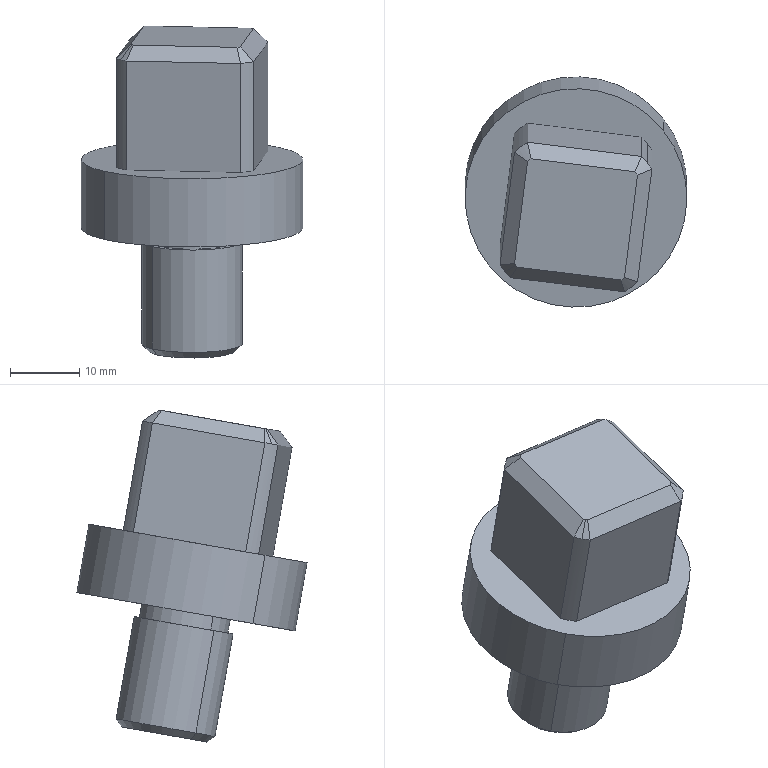Component | SolidWorks | 27PlugScrew-1 | 1 solid | 31 faces | box 32 x 33.25 x 47.93 mm | volume 17888 mm3 | plane 13 | cylinder 11 | cone 7 | commonest cylinder face diameters 26 x5 14.5 x2 13 x2 32 x2
STEP:
#1=COLOUR_RGB('',0.7922,0.8196,0.9333);
#2=FILL_AREA_STYLE_COLOUR('',#1);
#3=FILL_AREA_STYLE('',(#2));
#4=SURFACE_STYLE_FILL_AREA(#3);
#5=SURFACE_SIDE_STYLE('',(#4));
#6=SURFACE_STYLE_USAGE(.BOTH.,#5);
#7=PRESENTATION_STYLE_ASSIGNMENT((#6));
#8=CARTESIAN_POINT('',(2.951,-7.079,23.));
#9=VERTEX_POINT('',#8);
#10=CARTESIAN_POINT('',(3.339,-6.782,23.053));
#11=VERTEX_POINT('',#10);
#12=CARTESIAN_POINT('',(3.145,-6.931,23.027));
#13=DIRECTION('',(-0.,0.1736,-0.9848));
#14=DIRECTION('',(-0.7898,-0.6041,-0.1065));
#15=AXIS2_PLACEMENT_3D('',#12,#13,#14);
#16=CIRCLE('',#15,0.2461);
#17=EDGE_CURVE('',#9,#11,#16,.T.);
#18=ORIENTED_EDGE('',*,*,#17,.F.);
#19=CARTESIAN_POINT('',(2.92,-7.11,23.035));
#20=VERTEX_POINT('',#19);
#21=CARTESIAN_POINT('',(2.951,-7.079,23.));
#22=DIRECTION('',(-0.5585,-0.5499,0.621));
#23=VECTOR('',#22,39.37);
#24=LINE('',#21,#23);
#25=EDGE_CURVE('',#9,#20,#24,.T.);
#26=ORIENTED_EDGE('',*,*,#25,.T.);
#27=CARTESIAN_POINT('',(3.37,-6.765,23.096));
#28=VERTEX_POINT('',#27);
#29=CARTESIAN_POINT('',(3.145,-6.938,23.065));
#30=DIRECTION('',(0.,-0.1736,0.9848));
#31=DIRECTION('',(-0.7898,-0.6041,-0.1065));
#32=AXIS2_PLACEMENT_3D('',#29,#30,#31);
#33=CIRCLE('',#32,0.2854);
#34=EDGE_CURVE('',#28,#20,#33,.T.);
#35=ORIENTED_EDGE('',*,*,#34,.F.);
#36=CARTESIAN_POINT('',(3.339,-6.782,23.053));
#37=DIRECTION('',(0.5585,0.3043,0.7717));
#38=VECTOR('',#37,39.37);
#39=LINE('',#36,#38);
#40=EDGE_CURVE('',#11,#28,#39,.T.);
#41=ORIENTED_EDGE('',*,*,#40,.F.);
#42=EDGE_LOOP('',(#18,#26,#35,#41));
#43=FACE_OUTER_BOUND('',#42,.T.);
#44=CARTESIAN_POINT('',(3.145,-6.931,23.027));
#45=DIRECTION('',(0.,-0.1736,0.9848));
#46=DIRECTION('',(0.7898,0.6041,0.1065));
#47=AXIS2_PLACEMENT_3D('',#44,#45,#46);
#48=CONICAL_SURFACE('',#47,0.2461,0.7854);
#49=ADVANCED_FACE('',(#43),#48,.T.);
#50=CARTESIAN_POINT('',(2.803,-7.507,24.764));
#51=VERTEX_POINT('',#50);
#52=CARTESIAN_POINT('',(2.811,-7.516,24.762));
#53=VERTEX_POINT('',#52);
#54=CARTESIAN_POINT('',(3.145,-7.245,24.81));
#55=DIRECTION('',(0.,-0.1736,0.9848));
#56=DIRECTION('',(-0.7898,-0.6041,-0.1065));
#57=AXIS2_PLACEMENT_3D('',#54,#55,#56);
#58=CIRCLE('',#57,0.4331);
#59=EDGE_CURVE('',#51,#53,#58,.T.);
#60=ORIENTED_EDGE('',*,*,#59,.F.);
#61=CARTESIAN_POINT('',(2.741,-7.541,24.678));
#62=VERTEX_POINT('',#61);
#63=CARTESIAN_POINT('',(2.741,-7.541,24.678));
#64=DIRECTION('',(-0.5585,-0.3043,-0.7717));
#65=VECTOR('',#64,39.37);
#66=LINE('',#63,#65);
#67=EDGE_CURVE('',#51,#62,#66,.T.);
#68=ORIENTED_EDGE('',*,*,#67,.T.);
#69=CARTESIAN_POINT('',(2.771,-7.576,24.672));
#70=VERTEX_POINT('',#69);
#71=CARTESIAN_POINT('',(3.145,-7.232,24.733));
#72=DIRECTION('',(-0.,0.1736,-0.9848));
#73=DIRECTION('',(-0.7898,-0.6041,-0.1065));
#74=AXIS2_PLACEMENT_3D('',#71,#72,#73);
#75=CIRCLE('',#74,0.5118);
#76=EDGE_CURVE('',#70,#62,#75,.T.);
#77=ORIENTED_EDGE('',*,*,#76,.F.);
#78=CARTESIAN_POINT('',(2.771,-7.576,24.672));
#79=CARTESIAN_POINT('',(2.784,-7.556,24.702));
#80=CARTESIAN_POINT('',(2.797,-7.536,24.732));
#81=CARTESIAN_POINT('',(2.811,-7.516,24.762));
#82=B_SPLINE_CURVE_WITH_KNOTS('',3,(#78,#79,#80,#81),.UNSPECIFIED.,.F.,.F.,(4,4),(0.,0.002928),.UNSPECIFIED.);
#83=EDGE_CURVE('',#70,#53,#82,.T.);
#84=ORIENTED_EDGE('',*,*,#83,.T.);
#85=EDGE_LOOP('',(#60,#68,#77,#84));
#86=FACE_OUTER_BOUND('',#85,.T.);
#87=CARTESIAN_POINT('',(3.145,-7.232,24.733));
#88=DIRECTION('',(-0.,0.1736,-0.9848));
#89=DIRECTION('',(-0.7898,-0.6041,-0.1065));
#90=AXIS2_PLACEMENT_3D('',#87,#88,#89);
#91=CONICAL_SURFACE('',#90,0.5118,0.7854);
#92=ADVANCED_FACE('',(#86),#91,.T.);
#93=ORIENTED_EDGE('',*,*,#34,.T.);
#94=CARTESIAN_POINT('',(2.92,-7.213,23.617));
#95=VERTEX_POINT('',#94);
#96=CARTESIAN_POINT('',(2.92,-7.103,22.996));
#97=DIRECTION('',(0.,-0.1736,0.9848));
#98=VECTOR('',#97,39.37);
#99=LINE('',#96,#98);
#100=EDGE_CURVE('',#20,#95,#99,.T.);
#101=ORIENTED_EDGE('',*,*,#100,.T.);
#102=CARTESIAN_POINT('',(3.37,-6.868,23.677));
#103=VERTEX_POINT('',#102);
#104=CARTESIAN_POINT('',(3.145,-7.04,23.647));
#105=DIRECTION('',(-0.,0.1736,-0.9848));
#106=DIRECTION('',(-0.7898,-0.6041,-0.1065));
#107=AXIS2_PLACEMENT_3D('',#104,#105,#106);
#108=CIRCLE('',#107,0.2854);
#109=EDGE_CURVE('',#95,#103,#108,.T.);
#110=ORIENTED_EDGE('',*,*,#109,.T.);
#111=CARTESIAN_POINT('',(3.37,-6.758,23.057));
#112=DIRECTION('',(0.,-0.1736,0.9848));
#113=VECTOR('',#112,39.37);
#114=LINE('',#111,#113);
#115=EDGE_CURVE('',#28,#103,#114,.T.);
#116=ORIENTED_EDGE('',*,*,#115,.F.);
#117=EDGE_LOOP('',(#93,#101,#110,#116));
#118=FACE_OUTER_BOUND('',#117,.T.);
#119=CARTESIAN_POINT('',(3.145,-6.931,23.027));
#120=DIRECTION('',(0.,-0.1736,0.9848));
#121=DIRECTION('',(0.7898,0.6041,0.1065));
#122=AXIS2_PLACEMENT_3D('',#119,#120,#121);
#123=CYLINDRICAL_SURFACE('',#122,0.2854);
#124=ADVANCED_FACE('',(#118),#123,.T.);
#125=CARTESIAN_POINT('',(2.943,-7.195,23.62));
#126=VERTEX_POINT('',#125);
#127=CARTESIAN_POINT('',(3.347,-6.886,23.674));
#128=VERTEX_POINT('',#127);
#129=CARTESIAN_POINT('',(3.145,-7.04,23.647));
#130=DIRECTION('',(-0.,0.1736,-0.9848));
#131=DIRECTION('',(-0.7898,-0.6041,-0.1065));
#132=AXIS2_PLACEMENT_3D('',#129,#130,#131);
#133=CIRCLE('',#132,0.2559);
#134=EDGE_CURVE('',#126,#128,#133,.T.);
#135=ORIENTED_EDGE('',*,*,#134,.F.);
#136=CARTESIAN_POINT('',(2.943,-7.208,23.697));
#137=VERTEX_POINT('',#136);
#138=CARTESIAN_POINT('',(2.943,-7.195,23.62));
#139=DIRECTION('',(0.,-0.1736,0.9848));
#140=VECTOR('',#139,39.37);
#141=LINE('',#138,#140);
#142=EDGE_CURVE('',#126,#137,#141,.T.);
#143=ORIENTED_EDGE('',*,*,#142,.T.);
#144=CARTESIAN_POINT('',(3.347,-6.899,23.752));
#145=VERTEX_POINT('',#144);
#146=CARTESIAN_POINT('',(3.145,-7.054,23.725));
#147=DIRECTION('',(-0.,0.1736,-0.9848));
#148=DIRECTION('',(-0.7898,-0.6041,-0.1065));
#149=AXIS2_PLACEMENT_3D('',#146,#147,#148);
#150=CIRCLE('',#149,0.2559);
#151=EDGE_CURVE('',#137,#145,#150,.T.);
#152=ORIENTED_EDGE('',*,*,#151,.T.);
#153=CARTESIAN_POINT('',(3.347,-6.886,23.674));
#154=DIRECTION('',(0.,-0.1736,0.9848));
#155=VECTOR('',#154,39.37);
#156=LINE('',#153,#155);
#157=EDGE_CURVE('',#128,#145,#156,.T.);
#158=ORIENTED_EDGE('',*,*,#157,.F.);
#159=EDGE_LOOP('',(#135,#143,#152,#158));
#160=FACE_OUTER_BOUND('',#159,.T.);
#161=CARTESIAN_POINT('',(3.145,-7.04,23.647));
#162=DIRECTION('',(0.,-0.1736,0.9848));
#163=DIRECTION('',(0.7898,0.6041,0.1065));
#164=AXIS2_PLACEMENT_3D('',#161,#162,#163);
#165=CYLINDRICAL_SURFACE('',#164,0.2559);
#166=ADVANCED_FACE('',(#160),#165,.T.);
#167=CARTESIAN_POINT('',(2.648,-7.434,23.657));
#168=VERTEX_POINT('',#167);
#169=CARTESIAN_POINT('',(3.643,-6.673,23.792));
#170=VERTEX_POINT('',#169);
#171=CARTESIAN_POINT('',(3.145,-7.054,23.725));
#172=DIRECTION('',(-0.,0.1736,-0.9848));
#173=DIRECTION('',(-0.7898,-0.6041,-0.1065));
#174=AXIS2_PLACEMENT_3D('',#171,#172,#173);
#175=CIRCLE('',#174,0.6299);
#176=EDGE_CURVE('',#168,#170,#175,.T.);
#177=ORIENTED_EDGE('',*,*,#176,.F.);
#178=CARTESIAN_POINT('',(2.648,-7.503,24.045));
#179=VERTEX_POINT('',#178);
#180=CARTESIAN_POINT('',(2.648,-7.434,23.657));
#181=DIRECTION('',(0.,-0.1736,0.9848));
#182=VECTOR('',#181,39.37);
#183=LINE('',#180,#182);
#184=EDGE_CURVE('',#168,#179,#183,.T.);
#185=ORIENTED_EDGE('',*,*,#184,.T.);
#186=CARTESIAN_POINT('',(3.643,-6.742,24.179));
#187=VERTEX_POINT('',#186);
#188=CARTESIAN_POINT('',(3.145,-7.122,24.112));
#189=DIRECTION('',(-0.,0.1736,-0.9848));
#190=DIRECTION('',(-0.7898,-0.6041,-0.1065));
#191=AXIS2_PLACEMENT_3D('',#188,#189,#190);
#192=CIRCLE('',#191,0.6299);
#193=EDGE_CURVE('',#179,#187,#192,.T.);
#194=ORIENTED_EDGE('',*,*,#193,.T.);
#195=CARTESIAN_POINT('',(3.643,-6.673,23.792));
#196=DIRECTION('',(0.,-0.1736,0.9848));
#197=VECTOR('',#196,39.37);
#198=LINE('',#195,#197);
#199=EDGE_CURVE('',#170,#187,#198,.T.);
#200=ORIENTED_EDGE('',*,*,#199,.F.);
#201=EDGE_LOOP('',(#177,#185,#194,#200));
#202=FACE_OUTER_BOUND('',#201,.T.);
#203=CARTESIAN_POINT('',(3.145,-7.054,23.725));
#204=DIRECTION('',(0.,-0.1736,0.9848));
#205=DIRECTION('',(0.7898,0.6041,0.1065));
#206=AXIS2_PLACEMENT_3D('',#203,#204,#205);
#207=CYLINDRICAL_SURFACE('',#206,0.6299);
#208=ADVANCED_FACE('',(#202),#207,.T.);
#209=CARTESIAN_POINT('',(3.549,-6.813,24.167));
#210=VERTEX_POINT('',#209);
#211=CARTESIAN_POINT('',(3.576,-6.851,24.16));
#212=VERTEX_POINT('',#211);
#213=CARTESIAN_POINT('',(3.145,-7.122,24.112));
#214=DIRECTION('',(-0.,0.1736,-0.9848));
#215=DIRECTION('',(-0.7898,-0.6041,-0.1065));
#216=AXIS2_PLACEMENT_3D('',#213,#214,#215);
#217=CIRCLE('',#216,0.5118);
#218=EDGE_CURVE('',#210,#212,#217,.T.);
#219=ORIENTED_EDGE('',*,*,#218,.F.);
#220=CARTESIAN_POINT('',(3.549,-6.922,24.787));
#221=VERTEX_POINT('',#220);
#222=CARTESIAN_POINT('',(3.549,-6.813,24.167));
#223=DIRECTION('',(0.,-0.1736,0.9848));
#224=VECTOR('',#223,39.37);
#225=LINE('',#222,#224);
#226=EDGE_CURVE('',#210,#221,#225,.T.);
#227=ORIENTED_EDGE('',*,*,#226,.T.);
#228=CARTESIAN_POINT('',(3.576,-6.96,24.78));
#229=VERTEX_POINT('',#228);
#230=CARTESIAN_POINT('',(3.145,-7.232,24.733));
#231=DIRECTION('',(-0.,0.1736,-0.9848));
#232=DIRECTION('',(-0.7898,-0.6041,-0.1065));
#233=AXIS2_PLACEMENT_3D('',#230,#231,#232);
#234=CIRCLE('',#233,0.5118);
#235=EDGE_CURVE('',#221,#229,#234,.T.);
#236=ORIENTED_EDGE('',*,*,#235,.T.);
#237=CARTESIAN_POINT('',(3.576,-6.851,24.16));
#238=DIRECTION('',(0.,-0.1736,0.9848));
#239=VECTOR('',#238,39.37);
#240=LINE('',#237,#239);
#241=EDGE_CURVE('',#212,#229,#240,.T.);
#242=ORIENTED_EDGE('',*,*,#241,.F.);
#243=EDGE_LOOP('',(#219,#227,#236,#242));
#244=FACE_OUTER_BOUND('',#243,.T.);
#245=CARTESIAN_POINT('',(3.145,-7.122,24.112));
#246=DIRECTION('',(0.,-0.1736,0.9848));
#247=DIRECTION('',(0.7898,0.6041,0.1065));
#248=AXIS2_PLACEMENT_3D('',#245,#246,#247);
#249=CYLINDRICAL_SURFACE('',#248,0.5118);
#250=ADVANCED_FACE('',(#244),#249,.T.);
#251=CARTESIAN_POINT('',(2.795,-6.754,24.177));
#252=VERTEX_POINT('',#251);
#253=CARTESIAN_POINT('',(2.795,-6.864,24.797));
#254=VERTEX_POINT('',#253);
#255=CARTESIAN_POINT('',(2.795,-6.754,24.177));
#256=DIRECTION('',(0.,-0.1736,0.9848));
#257=VECTOR('',#256,39.37);
#258=LINE('',#255,#257);
#259=EDGE_CURVE('',#252,#254,#258,.T.);
#260=ORIENTED_EDGE('',*,*,#259,.T.);
#261=CARTESIAN_POINT('',(2.87,-6.807,24.807));
#262=VERTEX_POINT('',#261);
#263=CARTESIAN_POINT('',(3.145,-7.232,24.733));
#264=DIRECTION('',(-0.,0.1736,-0.9848));
#265=DIRECTION('',(-0.7898,-0.6041,-0.1065));
#266=AXIS2_PLACEMENT_3D('',#263,#264,#265);
#267=CIRCLE('',#266,0.5118);
#268=EDGE_CURVE('',#254,#262,#267,.T.);
#269=ORIENTED_EDGE('',*,*,#268,.T.);
#270=CARTESIAN_POINT('',(2.87,-6.697,24.187));
#271=VERTEX_POINT('',#270);
#272=CARTESIAN_POINT('',(2.87,-6.697,24.187));
#273=DIRECTION('',(0.,-0.1736,0.9848));
#274=VECTOR('',#273,39.37);
#275=LINE('',#272,#274);
#276=EDGE_CURVE('',#271,#262,#275,.T.);
#277=ORIENTED_EDGE('',*,*,#276,.F.);
#278=CARTESIAN_POINT('',(3.145,-7.122,24.112));
#279=DIRECTION('',(-0.,0.1736,-0.9848));
#280=DIRECTION('',(-0.7898,-0.6041,-0.1065));
#281=AXIS2_PLACEMENT_3D('',#278,#279,#280);
#282=CIRCLE('',#281,0.5118);
#283=EDGE_CURVE('',#252,#271,#282,.T.);
#284=ORIENTED_EDGE('',*,*,#283,.F.);
#285=EDGE_LOOP('',(#260,#269,#277,#284));
#286=FACE_OUTER_BOUND('',#285,.T.);
#287=CARTESIAN_POINT('',(3.145,-7.122,24.112));
#288=DIRECTION('',(0.,-0.1736,0.9848));
#289=DIRECTION('',(0.7898,0.6041,0.1065));
#290=AXIS2_PLACEMENT_3D('',#287,#288,#289);
#291=CYLINDRICAL_SURFACE('',#290,0.5118);
#292=ADVANCED_FACE('',(#286),#291,.T.);
#293=ORIENTED_EDGE('',*,*,#276,.T.);
#294=CARTESIAN_POINT('',(3.519,-6.887,24.793));
#295=VERTEX_POINT('',#294);
#296=CARTESIAN_POINT('',(2.87,-6.807,24.807));
#297=DIRECTION('',(0.9922,-0.1228,-0.02166));
#298=VECTOR('',#297,39.37);
#299=LINE('',#296,#298);
#300=EDGE_CURVE('',#262,#295,#299,.T.);
#301=ORIENTED_EDGE('',*,*,#300,.T.);
#302=CARTESIAN_POINT('',(3.519,-6.778,24.173));
#303=VERTEX_POINT('',#302);
#304=CARTESIAN_POINT('',(3.519,-6.778,24.173));
#305=DIRECTION('',(0.,-0.1736,0.9848));
#306=VECTOR('',#305,39.37);
#307=LINE('',#304,#306);
#308=EDGE_CURVE('',#303,#295,#307,.T.);
#309=ORIENTED_EDGE('',*,*,#308,.F.);
#310=CARTESIAN_POINT('',(2.87,-6.697,24.187));
#311=DIRECTION('',(0.9922,-0.1228,-0.02166));
#312=VECTOR('',#311,39.37);
#313=LINE('',#310,#312);
#314=EDGE_CURVE('',#271,#303,#313,.T.);
#315=ORIENTED_EDGE('',*,*,#314,.F.);
#316=EDGE_LOOP('',(#293,#301,#309,#315));
#317=FACE_OUTER_BOUND('',#316,.T.);
#318=CARTESIAN_POINT('',(2.87,-6.697,24.187));
#319=DIRECTION('',(-0.1247,-0.9771,-0.1723));
#320=DIRECTION('',(-0.9922,0.1228,0.02166));
#321=AXIS2_PLACEMENT_3D('',#318,#319,#320);
#322=PLANE('',#321);
#323=ADVANCED_FACE('',(#317),#322,.F.);
#324=ORIENTED_EDGE('',*,*,#226,.F.);
#325=CARTESIAN_POINT('',(3.145,-7.122,24.112));
#326=DIRECTION('',(-0.,0.1736,-0.9848));
#327=DIRECTION('',(-0.7898,-0.6041,-0.1065));
#328=AXIS2_PLACEMENT_3D('',#325,#326,#327);
#329=CIRCLE('',#328,0.5118);
#330=EDGE_CURVE('',#303,#210,#329,.T.);
#331=ORIENTED_EDGE('',*,*,#330,.F.);
#332=ORIENTED_EDGE('',*,*,#308,.T.);
#333=CARTESIAN_POINT('',(3.145,-7.232,24.733));
#334=DIRECTION('',(-0.,0.1736,-0.9848));
#335=DIRECTION('',(-0.7898,-0.6041,-0.1065));
#336=AXIS2_PLACEMENT_3D('',#333,#334,#335);
#337=CIRCLE('',#336,0.5118);
#338=EDGE_CURVE('',#295,#221,#337,.T.);
#339=ORIENTED_EDGE('',*,*,#338,.T.);
#340=EDGE_LOOP('',(#324,#331,#332,#339));
#341=FACE_OUTER_BOUND('',#340,.T.);
#342=CARTESIAN_POINT('',(3.145,-7.122,24.112));
#343=DIRECTION('',(0.,-0.1736,0.9848));
#344=DIRECTION('',(0.7898,0.6041,0.1065));
#345=AXIS2_PLACEMENT_3D('',#342,#343,#344);
#346=CYLINDRICAL_SURFACE('',#345,0.5118);
#347=ADVANCED_FACE('',(#341),#346,.T.);
#348=ORIENTED_EDGE('',*,*,#241,.T.);
#349=CARTESIAN_POINT('',(3.495,-7.599,24.668));
#350=VERTEX_POINT('',#349);
#351=CARTESIAN_POINT('',(3.495,-7.599,24.668));
#352=DIRECTION('',(-0.1247,-0.9771,-0.1723));
#353=VECTOR('',#352,39.37);
#354=LINE('',#351,#353);
#355=EDGE_CURVE('',#229,#350,#354,.T.);
#356=ORIENTED_EDGE('',*,*,#355,.T.);
#357=CARTESIAN_POINT('',(3.495,-7.49,24.047));
#358=VERTEX_POINT('',#357);
#359=CARTESIAN_POINT('',(3.495,-7.49,24.047));
#360=DIRECTION('',(0.,-0.1736,0.9848));
#361=VECTOR('',#360,39.37);
#362=LINE('',#359,#361);
#363=EDGE_CURVE('',#358,#350,#362,.T.);
#364=ORIENTED_EDGE('',*,*,#363,.F.);
#365=CARTESIAN_POINT('',(3.495,-7.49,24.047));
#366=DIRECTION('',(-0.1247,-0.9771,-0.1723));
#367=VECTOR('',#366,39.37);
#368=LINE('',#365,#367);
#369=EDGE_CURVE('',#212,#358,#368,.T.);
#370=ORIENTED_EDGE('',*,*,#369,.F.);
#371=EDGE_LOOP('',(#348,#356,#364,#370));
#372=FACE_OUTER_BOUND('',#371,.T.);
#373=CARTESIAN_POINT('',(3.495,-7.49,24.047));
#374=DIRECTION('',(-0.9922,0.1228,0.02166));
#375=DIRECTION('',(0.1247,0.9771,0.1723));
#376=AXIS2_PLACEMENT_3D('',#373,#374,#375);
#377=PLANE('',#376);
#378=ADVANCED_FACE('',(#372),#377,.F.);
#379=ORIENTED_EDGE('',*,*,#363,.T.);
#380=CARTESIAN_POINT('',(3.42,-7.656,24.658));
#381=VERTEX_POINT('',#380);
#382=CARTESIAN_POINT('',(3.145,-7.232,24.733));
#383=DIRECTION('',(-0.,0.1736,-0.9848));
#384=DIRECTION('',(-0.7898,-0.6041,-0.1065));
#385=AXIS2_PLACEMENT_3D('',#382,#383,#384);
#386=CIRCLE('',#385,0.5118);
#387=EDGE_CURVE('',#350,#381,#386,.T.);
#388=ORIENTED_EDGE('',*,*,#387,.T.);
#389=CARTESIAN_POINT('',(3.42,-7.547,24.037));
#390=VERTEX_POINT('',#389);
#391=CARTESIAN_POINT('',(3.42,-7.547,24.037));
#392=DIRECTION('',(0.,-0.1736,0.9848));
#393=VECTOR('',#392,39.37);
#394=LINE('',#391,#393);
#395=EDGE_CURVE('',#390,#381,#394,.T.);
#396=ORIENTED_EDGE('',*,*,#395,.F.);
#397=CARTESIAN_POINT('',(3.145,-7.122,24.112));
#398=DIRECTION('',(-0.,0.1736,-0.9848));
#399=DIRECTION('',(-0.7898,-0.6041,-0.1065));
#400=AXIS2_PLACEMENT_3D('',#397,#398,#399);
#401=CIRCLE('',#400,0.5118);
#402=EDGE_CURVE('',#358,#390,#401,.T.);
#403=ORIENTED_EDGE('',*,*,#402,.F.);
#404=EDGE_LOOP('',(#379,#388,#396,#403));
#405=FACE_OUTER_BOUND('',#404,.T.);
#406=CARTESIAN_POINT('',(3.145,-7.122,24.112));
#407=DIRECTION('',(0.,-0.1736,0.9848));
#408=DIRECTION('',(0.7898,0.6041,0.1065));
#409=AXIS2_PLACEMENT_3D('',#406,#407,#408);
#410=CYLINDRICAL_SURFACE('',#409,0.5118);
#411=ADVANCED_FACE('',(#405),#410,.T.);
#412=ORIENTED_EDGE('',*,*,#395,.T.);
#413=CARTESIAN_POINT('',(3.42,-7.656,24.658));
#414=DIRECTION('',(-0.9922,0.1228,0.02166));
#415=VECTOR('',#414,39.37);
#416=LINE('',#413,#415);
#417=EDGE_CURVE('',#381,#70,#416,.T.);
#418=ORIENTED_EDGE('',*,*,#417,.T.);
#419=CARTESIAN_POINT('',(2.771,-7.467,24.051));
#420=VERTEX_POINT('',#419);
#421=CARTESIAN_POINT('',(2.771,-7.467,24.051));
#422=DIRECTION('',(0.,-0.1736,0.9848));
#423=VECTOR('',#422,39.37);
#424=LINE('',#421,#423);
#425=EDGE_CURVE('',#420,#70,#424,.T.);
#426=ORIENTED_EDGE('',*,*,#425,.F.);
#427=CARTESIAN_POINT('',(3.42,-7.547,24.037));
#428=DIRECTION('',(-0.9922,0.1228,0.02166));
#429=VECTOR('',#428,39.37);
#430=LINE('',#427,#429);
#431=EDGE_CURVE('',#390,#420,#430,.T.);
#432=ORIENTED_EDGE('',*,*,#431,.F.);
#433=EDGE_LOOP('',(#412,#418,#426,#432));
#434=FACE_OUTER_BOUND('',#433,.T.);
#435=CARTESIAN_POINT('',(3.42,-7.547,24.037));
#436=DIRECTION('',(0.1247,0.9771,0.1723));
#437=DIRECTION('',(0.9922,-0.1228,-0.02166));
#438=AXIS2_PLACEMENT_3D('',#435,#436,#437);
#439=PLANE('',#438);
#440=ADVANCED_FACE('',(#434),#439,.F.);
#441=ORIENTED_EDGE('',*,*,#425,.T.);
#442=ORIENTED_EDGE('',*,*,#76,.T.);
#443=CARTESIAN_POINT('',(2.714,-7.503,24.685));
#444=VERTEX_POINT('',#443);
#445=CARTESIAN_POINT('',(3.145,-7.232,24.733));
#446=DIRECTION('',(-0.,0.1736,-0.9848));
#447=DIRECTION('',(-0.7898,-0.6041,-0.1065));
#448=AXIS2_PLACEMENT_3D('',#445,#446,#447);
#449=CIRCLE('',#448,0.5118);
#450=EDGE_CURVE('',#62,#444,#449,.T.);
#451=ORIENTED_EDGE('',*,*,#450,.T.);
#452=CARTESIAN_POINT('',(2.714,-7.393,24.064));
#453=VERTEX_POINT('',#452);
#454=CARTESIAN_POINT('',(2.714,-7.393,24.064));
#455=DIRECTION('',(0.,-0.1736,0.9848));
#456=VECTOR('',#455,39.37);
#457=LINE('',#454,#456);
#458=EDGE_CURVE('',#453,#444,#457,.T.);
#459=ORIENTED_EDGE('',*,*,#458,.F.);
#460=CARTESIAN_POINT('',(3.145,-7.122,24.112));
#461=DIRECTION('',(-0.,0.1736,-0.9848));
#462=DIRECTION('',(-0.7898,-0.6041,-0.1065));
#463=AXIS2_PLACEMENT_3D('',#460,#461,#462);
#464=CIRCLE('',#463,0.5118);
#465=EDGE_CURVE('',#420,#453,#464,.T.);
#466=ORIENTED_EDGE('',*,*,#465,.F.);
#467=EDGE_LOOP('',(#441,#442,#451,#459,#466));
#468=FACE_OUTER_BOUND('',#467,.T.);
#469=CARTESIAN_POINT('',(3.145,-7.122,24.112));
#470=DIRECTION('',(0.,-0.1736,0.9848));
#471=DIRECTION('',(0.7898,0.6041,0.1065));
#472=AXIS2_PLACEMENT_3D('',#469,#470,#471);
#473=CYLINDRICAL_SURFACE('',#472,0.5118);
#474=ADVANCED_FACE('',(#468),#473,.T.);
#475=ORIENTED_EDGE('',*,*,#458,.T.);
#476=CARTESIAN_POINT('',(2.795,-6.864,24.797));
#477=DIRECTION('',(0.1247,0.9771,0.1723));
#478=VECTOR('',#477,39.37);
#479=LINE('',#476,#478);
#480=EDGE_CURVE('',#444,#254,#479,.T.);
#481=ORIENTED_EDGE('',*,*,#480,.T.);
#482=ORIENTED_EDGE('',*,*,#259,.F.);
#483=CARTESIAN_POINT('',(2.795,-6.754,24.177));
#484=DIRECTION('',(0.1247,0.9771,0.1723));
#485=VECTOR('',#484,39.37);
#486=LINE('',#483,#485);
#487=EDGE_CURVE('',#453,#252,#486,.T.);
#488=ORIENTED_EDGE('',*,*,#487,.F.);
#489=EDGE_LOOP('',(#475,#481,#482,#488));
#490=FACE_OUTER_BOUND('',#489,.T.);
#491=CARTESIAN_POINT('',(2.795,-6.754,24.177));
#492=DIRECTION('',(0.9922,-0.1228,-0.02166));
#493=DIRECTION('',(-0.1247,-0.9771,-0.1723));
#494=AXIS2_PLACEMENT_3D('',#491,#492,#493);
#495=PLANE('',#494);
#496=ADVANCED_FACE('',(#490),#495,.F.);
#497=CARTESIAN_POINT('',(3.495,-6.993,24.855));
#498=VERTEX_POINT('',#497);
#499=CARTESIAN_POINT('',(3.479,-6.974,24.858));
#500=VERTEX_POINT('',#499);
#501=CARTESIAN_POINT('',(3.145,-7.245,24.81));
#502=DIRECTION('',(0.,-0.1736,0.9848));
#503=DIRECTION('',(-0.7898,-0.6041,-0.1065));
#504=AXIS2_PLACEMENT_3D('',#501,#502,#503);
#505=CIRCLE('',#504,0.4331);
#506=EDGE_CURVE('',#498,#500,#505,.T.);
#507=ORIENTED_EDGE('',*,*,#506,.T.);
#508=CARTESIAN_POINT('',(2.889,-6.901,24.871));
#509=VERTEX_POINT('',#508);
#510=CARTESIAN_POINT('',(3.184,-6.937,24.864));
#511=DIRECTION('',(-0.9922,0.1228,0.02166));
#512=VECTOR('',#511,39.37);
#513=LINE('',#510,#512);
#514=EDGE_CURVE('',#500,#509,#513,.T.);
#515=ORIENTED_EDGE('',*,*,#514,.T.);
#516=CARTESIAN_POINT('',(2.87,-6.916,24.868));
#517=VERTEX_POINT('',#516);
#518=CARTESIAN_POINT('',(3.145,-7.245,24.81));
#519=DIRECTION('',(0.,-0.1736,0.9848));
#520=DIRECTION('',(-0.7898,-0.6041,-0.1065));
#521=AXIS2_PLACEMENT_3D('',#518,#519,#520);
#522=CIRCLE('',#521,0.4331);
#523=EDGE_CURVE('',#509,#517,#522,.T.);
#524=ORIENTED_EDGE('',*,*,#523,.T.);
#525=CARTESIAN_POINT('',(2.795,-7.497,24.766));
#526=VERTEX_POINT('',#525);
#527=CARTESIAN_POINT('',(2.833,-7.207,24.817));
#528=DIRECTION('',(-0.1247,-0.9771,-0.1723));
#529=VECTOR('',#528,39.37);
#530=LINE('',#527,#529);
#531=EDGE_CURVE('',#517,#526,#530,.T.);
#532=ORIENTED_EDGE('',*,*,#531,.T.);
#533=CARTESIAN_POINT('',(3.145,-7.245,24.81));
#534=DIRECTION('',(0.,-0.1736,0.9848));
#535=DIRECTION('',(-0.7898,-0.6041,-0.1065));
#536=AXIS2_PLACEMENT_3D('',#533,#534,#535);
#537=CIRCLE('',#536,0.4331);
#538=EDGE_CURVE('',#526,#51,#537,.T.);
#539=ORIENTED_EDGE('',*,*,#538,.T.);
#540=ORIENTED_EDGE('',*,*,#59,.T.);
#541=CARTESIAN_POINT('',(3.401,-7.589,24.749));
#542=VERTEX_POINT('',#541);
#543=CARTESIAN_POINT('',(3.106,-7.553,24.756));
#544=DIRECTION('',(0.9922,-0.1228,-0.02166));
#545=VECTOR('',#544,39.37);
#546=LINE('',#543,#545);
#547=EDGE_CURVE('',#53,#542,#546,.T.);
#548=ORIENTED_EDGE('',*,*,#547,.T.);
#549=CARTESIAN_POINT('',(3.42,-7.574,24.752));
#550=VERTEX_POINT('',#549);
#551=CARTESIAN_POINT('',(3.145,-7.245,24.81));
#552=DIRECTION('',(0.,-0.1736,0.9848));
#553=DIRECTION('',(-0.7898,-0.6041,-0.1065));
#554=AXIS2_PLACEMENT_3D('',#551,#552,#553);
#555=CIRCLE('',#554,0.4331);
#556=EDGE_CURVE('',#542,#550,#555,.T.);
#557=ORIENTED_EDGE('',*,*,#556,.T.);
#558=CARTESIAN_POINT('',(3.458,-7.284,24.803));
#559=DIRECTION('',(0.1247,0.9771,0.1723));
#560=VECTOR('',#559,39.37);
#561=LINE('',#558,#560);
#562=EDGE_CURVE('',#550,#498,#561,.T.);
#563=ORIENTED_EDGE('',*,*,#562,.T.);
#564=EDGE_LOOP('',(#507,#515,#524,#532,#539,#540,#548,#557,#563));
#565=FACE_OUTER_BOUND('',#564,.T.);
#566=CARTESIAN_POINT('',(3.145,-7.245,24.81));
#567=DIRECTION('',(0.,0.1736,-0.9848));
#568=DIRECTION('',(-0.7898,-0.6041,-0.1065));
#569=AXIS2_PLACEMENT_3D('',#566,#567,#568);
#570=PLANE('',#569);
#571=ADVANCED_FACE('',(#565),#570,.F.);
#572=CARTESIAN_POINT('',(3.145,-7.122,24.112));
#573=DIRECTION('',(-0.,0.1736,-0.9848));
#574=DIRECTION('',(-0.7898,-0.6041,-0.1065));
#575=AXIS2_PLACEMENT_3D('',#572,#573,#574);
#576=CIRCLE('',#575,0.6299);
#577=EDGE_CURVE('',#187,#179,#576,.T.);
#578=ORIENTED_EDGE('',*,*,#577,.F.);
#579=ORIENTED_EDGE('',*,*,#193,.F.);
#580=EDGE_LOOP('',(#578,#579));
#581=FACE_OUTER_BOUND('',#580,.T.);
#582=ORIENTED_EDGE('',*,*,#487,.T.);
#583=ORIENTED_EDGE('',*,*,#283,.T.);
#584=ORIENTED_EDGE('',*,*,#314,.T.);
#585=ORIENTED_EDGE('',*,*,#330,.T.);
#586=ORIENTED_EDGE('',*,*,#218,.T.);
#587=ORIENTED_EDGE('',*,*,#369,.T.);
#588=ORIENTED_EDGE('',*,*,#402,.T.);
#589=ORIENTED_EDGE('',*,*,#431,.T.);
#590=ORIENTED_EDGE('',*,*,#465,.T.);
#591=EDGE_LOOP('',(#582,#583,#584,#585,#586,#587,#588,#589,#590));
#592=FACE_BOUND('',#591,.T.);
#593=CARTESIAN_POINT('',(3.145,-7.122,24.112));
#594=DIRECTION('',(0.,0.1736,-0.9848));
#595=DIRECTION('',(-0.7898,-0.6041,-0.1065));
#596=AXIS2_PLACEMENT_3D('',#593,#594,#595);
#597=PLANE('',#596);
#598=ADVANCED_FACE('',(#581,#592),#597,.F.);
#599=ORIENTED_EDGE('',*,*,#184,.F.);
#600=CARTESIAN_POINT('',(3.145,-7.054,23.725));
#601=DIRECTION('',(-0.,0.1736,-0.9848));
#602=DIRECTION('',(-0.7898,-0.6041,-0.1065));
#603=AXIS2_PLACEMENT_3D('',#600,#601,#602);
#604=CIRCLE('',#603,0.6299);
#605=EDGE_CURVE('',#170,#168,#604,.T.);
#606=ORIENTED_EDGE('',*,*,#605,.F.);
#607=ORIENTED_EDGE('',*,*,#199,.T.);
#608=ORIENTED_EDGE('',*,*,#577,.T.);
#609=EDGE_LOOP('',(#599,#606,#607,#608));
#610=FACE_OUTER_BOUND('',#609,.T.);
#611=CARTESIAN_POINT('',(3.145,-7.054,23.725));
#612=DIRECTION('',(0.,-0.1736,0.9848));
#613=DIRECTION('',(0.7898,0.6041,0.1065));
#614=AXIS2_PLACEMENT_3D('',#611,#612,#613);
#615=CYLINDRICAL_SURFACE('',#614,0.6299);
#616=ADVANCED_FACE('',(#610),#615,.T.);
#617=CARTESIAN_POINT('',(3.145,-7.054,23.725));
#618=DIRECTION('',(-0.,0.1736,-0.9848));
#619=DIRECTION('',(-0.7898,-0.6041,-0.1065));
#620=AXIS2_PLACEMENT_3D('',#617,#618,#619);
#621=CIRCLE('',#620,0.2559);
#622=EDGE_CURVE('',#145,#137,#621,.T.);
#623=ORIENTED_EDGE('',*,*,#622,.F.);
#624=ORIENTED_EDGE('',*,*,#151,.F.);
#625=EDGE_LOOP('',(#623,#624));
#626=FACE_BOUND('',#625,.T.);
#627=ORIENTED_EDGE('',*,*,#605,.T.);
#628=ORIENTED_EDGE('',*,*,#176,.T.);
#629=EDGE_LOOP('',(#627,#628));
#630=FACE_OUTER_BOUND('',#629,.T.);
#631=CARTESIAN_POINT('',(3.145,-7.054,23.725));
#632=DIRECTION('',(0.,0.1736,-0.9848));
#633=DIRECTION('',(-0.7898,-0.6041,-0.1065));
#634=AXIS2_PLACEMENT_3D('',#631,#632,#633);
#635=PLANE('',#634);
#636=ADVANCED_FACE('',(#626,#630),#635,.T.);
#637=ORIENTED_EDGE('',*,*,#142,.F.);
#638=CARTESIAN_POINT('',(3.145,-7.04,23.647));
#639=DIRECTION('',(-0.,0.1736,-0.9848));
#640=DIRECTION('',(-0.7898,-0.6041,-0.1065));
#641=AXIS2_PLACEMENT_3D('',#638,#639,#640);
#642=CIRCLE('',#641,0.2559);
#643=EDGE_CURVE('',#128,#126,#642,.T.);
#644=ORIENTED_EDGE('',*,*,#643,.F.);
#645=ORIENTED_EDGE('',*,*,#157,.T.);
#646=ORIENTED_EDGE('',*,*,#622,.T.);
#647=EDGE_LOOP('',(#637,#644,#645,#646));
#648=FACE_OUTER_BOUND('',#647,.T.);
#649=CARTESIAN_POINT('',(3.145,-7.04,23.647));
#650=DIRECTION('',(0.,-0.1736,0.9848));
#651=DIRECTION('',(0.7898,0.6041,0.1065));
#652=AXIS2_PLACEMENT_3D('',#649,#650,#651);
#653=CYLINDRICAL_SURFACE('',#652,0.2559);
#654=ADVANCED_FACE('',(#648),#653,.T.);
#655=ORIENTED_EDGE('',*,*,#100,.F.);
#656=CARTESIAN_POINT('',(3.145,-6.938,23.065));
#657=DIRECTION('',(0.,-0.1736,0.9848));
#658=DIRECTION('',(-0.7898,-0.6041,-0.1065));
#659=AXIS2_PLACEMENT_3D('',#656,#657,#658);
#660=CIRCLE('',#659,0.2854);
#661=EDGE_CURVE('',#20,#28,#660,.T.);
#662=ORIENTED_EDGE('',*,*,#661,.T.);
#663=ORIENTED_EDGE('',*,*,#115,.T.);
#664=CARTESIAN_POINT('',(3.145,-7.04,23.647));
#665=DIRECTION('',(-0.,0.1736,-0.9848));
#666=DIRECTION('',(-0.7898,-0.6041,-0.1065));
#667=AXIS2_PLACEMENT_3D('',#664,#665,#666);
#668=CIRCLE('',#667,0.2854);
#669=EDGE_CURVE('',#103,#95,#668,.T.);
#670=ORIENTED_EDGE('',*,*,#669,.T.);
#671=EDGE_LOOP('',(#655,#662,#663,#670));
#672=FACE_OUTER_BOUND('',#671,.T.);
#673=CARTESIAN_POINT('',(3.145,-6.931,23.027));
#674=DIRECTION('',(0.,-0.1736,0.9848));
#675=DIRECTION('',(0.7898,0.6041,0.1065));
#676=AXIS2_PLACEMENT_3D('',#673,#674,#675);
#677=CYLINDRICAL_SURFACE('',#676,0.2854);
#678=ADVANCED_FACE('',(#672),#677,.T.);
#679=CARTESIAN_POINT('',(3.145,-6.931,23.027));
#680=DIRECTION('',(-0.,0.1736,-0.9848));
#681=DIRECTION('',(-0.7898,-0.6041,-0.1065));
#682=AXIS2_PLACEMENT_3D('',#679,#680,#681);
#683=CIRCLE('',#682,0.2461);
#684=EDGE_CURVE('',#11,#9,#683,.T.);
#685=ORIENTED_EDGE('',*,*,#684,.T.);
#686=ORIENTED_EDGE('',*,*,#17,.T.);
#687=EDGE_LOOP('',(#685,#686));
#688=FACE_OUTER_BOUND('',#687,.T.);
#689=CARTESIAN_POINT('',(3.145,-6.931,23.027));
#690=DIRECTION('',(0.,0.1736,-0.9848));
#691=DIRECTION('',(-0.7898,-0.6041,-0.1065));
#692=AXIS2_PLACEMENT_3D('',#689,#690,#691);
#693=PLANE('',#692);
#694=ADVANCED_FACE('',(#688),#693,.T.);
#695=ORIENTED_EDGE('',*,*,#643,.T.);
#696=ORIENTED_EDGE('',*,*,#134,.T.);
#697=EDGE_LOOP('',(#695,#696));
#698=FACE_BOUND('',#697,.T.);
#699=ORIENTED_EDGE('',*,*,#669,.F.);
#700=ORIENTED_EDGE('',*,*,#109,.F.);
#701=EDGE_LOOP('',(#699,#700));
#702=FACE_OUTER_BOUND('',#701,.T.);
#703=CARTESIAN_POINT('',(3.145,-7.04,23.647));
#704=DIRECTION('',(0.,0.1736,-0.9848));
#705=DIRECTION('',(-0.7898,-0.6041,-0.1065));
#706=AXIS2_PLACEMENT_3D('',#703,#704,#705);
#707=PLANE('',#706);
#708=ADVANCED_FACE('',(#698,#702),#707,.F.);
#709=CARTESIAN_POINT('',(3.401,-7.589,24.749));
#710=CARTESIAN_POINT('',(3.408,-7.612,24.719));
#711=CARTESIAN_POINT('',(3.414,-7.634,24.688));
#712=CARTESIAN_POINT('',(3.42,-7.656,24.658));
#713=B_SPLINE_CURVE_WITH_KNOTS('',3,(#709,#710,#711,#712),.UNSPECIFIED.,.F.,.F.,(4,4),(0.,0.002928),.UNSPECIFIED.);
#714=EDGE_CURVE('',#542,#381,#713,.T.);
#715=ORIENTED_EDGE('',*,*,#714,.F.);
#716=ORIENTED_EDGE('',*,*,#547,.F.);
#717=ORIENTED_EDGE('',*,*,#83,.F.);
#718=ORIENTED_EDGE('',*,*,#417,.F.);
#719=EDGE_LOOP('',(#715,#716,#717,#718));
#720=FACE_OUTER_BOUND('',#719,.T.);
#721=CARTESIAN_POINT('',(3.42,-7.656,24.658));
#722=DIRECTION('',(0.08821,0.8137,-0.5745));
#723=DIRECTION('',(-0.9922,0.1228,0.02166));
#724=AXIS2_PLACEMENT_3D('',#721,#722,#723);
#725=PLANE('',#724);
#726=ADVANCED_FACE('',(#720),#725,.F.);
#727=ORIENTED_EDGE('',*,*,#67,.F.);
#728=ORIENTED_EDGE('',*,*,#538,.F.);
#729=CARTESIAN_POINT('',(2.714,-7.503,24.685));
#730=CARTESIAN_POINT('',(2.741,-7.501,24.712));
#731=CARTESIAN_POINT('',(2.768,-7.499,24.739));
#732=CARTESIAN_POINT('',(2.795,-7.497,24.766));
#733=B_SPLINE_CURVE_WITH_KNOTS('',3,(#729,#730,#731,#732),.UNSPECIFIED.,.F.,.F.,(4,4),(0.,0.002928),.UNSPECIFIED.);
#734=EDGE_CURVE('',#444,#526,#733,.T.);
#735=ORIENTED_EDGE('',*,*,#734,.F.);
#736=ORIENTED_EDGE('',*,*,#450,.F.);
#737=EDGE_LOOP('',(#727,#728,#735,#736));
#738=FACE_OUTER_BOUND('',#737,.T.);
#739=CARTESIAN_POINT('',(3.145,-7.232,24.733));
#740=DIRECTION('',(-0.,0.1736,-0.9848));
#741=DIRECTION('',(-0.7898,-0.6041,-0.1065));
#742=AXIS2_PLACEMENT_3D('',#739,#740,#741);
#743=CONICAL_SURFACE('',#742,0.5118,0.7854);
#744=ADVANCED_FACE('',(#738),#743,.T.);
#745=ORIENTED_EDGE('',*,*,#714,.T.);
#746=ORIENTED_EDGE('',*,*,#387,.F.);
#747=CARTESIAN_POINT('',(3.42,-7.574,24.752));
#748=CARTESIAN_POINT('',(3.445,-7.583,24.724));
#749=CARTESIAN_POINT('',(3.47,-7.592,24.696));
#750=CARTESIAN_POINT('',(3.495,-7.599,24.668));
#751=B_SPLINE_CURVE_WITH_KNOTS('',3,(#747,#748,#749,#750),.UNSPECIFIED.,.F.,.F.,(4,4),(0.,0.002928),.UNSPECIFIED.);
#752=EDGE_CURVE('',#550,#350,#751,.T.);
#753=ORIENTED_EDGE('',*,*,#752,.F.);
#754=ORIENTED_EDGE('',*,*,#556,.F.);
#755=EDGE_LOOP('',(#745,#746,#753,#754));
#756=FACE_OUTER_BOUND('',#755,.T.);
#757=CARTESIAN_POINT('',(3.145,-7.232,24.733));
#758=DIRECTION('',(-0.,0.1736,-0.9848));
#759=DIRECTION('',(-0.7898,-0.6041,-0.1065));
#760=AXIS2_PLACEMENT_3D('',#757,#758,#759);
#761=CONICAL_SURFACE('',#760,0.5118,0.7854);
#762=ADVANCED_FACE('',(#756),#761,.T.);
#763=ORIENTED_EDGE('',*,*,#734,.T.);
#764=ORIENTED_EDGE('',*,*,#531,.F.);
#765=CARTESIAN_POINT('',(2.795,-6.864,24.797));
#766=CARTESIAN_POINT('',(2.82,-6.881,24.821));
#767=CARTESIAN_POINT('',(2.845,-6.898,24.845));
#768=CARTESIAN_POINT('',(2.87,-6.916,24.868));
#769=B_SPLINE_CURVE_WITH_KNOTS('',3,(#765,#766,#767,#768),.UNSPECIFIED.,.F.,.F.,(4,4),(0.,0.002928),.UNSPECIFIED.);
#770=EDGE_CURVE('',#254,#517,#769,.T.);
#771=ORIENTED_EDGE('',*,*,#770,.F.);
#772=ORIENTED_EDGE('',*,*,#480,.F.);
#773=EDGE_LOOP('',(#763,#764,#771,#772));
#774=FACE_OUTER_BOUND('',#773,.T.);
#775=CARTESIAN_POINT('',(2.795,-6.864,24.797));
#776=DIRECTION('',(0.7016,0.03592,-0.7117));
#777=DIRECTION('',(0.1247,0.9771,0.1723));
#778=AXIS2_PLACEMENT_3D('',#775,#776,#777);
#779=PLANE('',#778);
#780=ADVANCED_FACE('',(#774),#779,.F.);
#781=ORIENTED_EDGE('',*,*,#752,.T.);
#782=ORIENTED_EDGE('',*,*,#355,.F.);
#783=CARTESIAN_POINT('',(3.495,-6.993,24.855));
#784=CARTESIAN_POINT('',(3.522,-6.982,24.83));
#785=CARTESIAN_POINT('',(3.549,-6.971,24.805));
#786=CARTESIAN_POINT('',(3.576,-6.96,24.78));
#787=B_SPLINE_CURVE_WITH_KNOTS('',3,(#783,#784,#785,#786),.UNSPECIFIED.,.F.,.F.,(4,4),(0.,0.002928),.UNSPECIFIED.);
#788=EDGE_CURVE('',#498,#229,#787,.T.);
#789=ORIENTED_EDGE('',*,*,#788,.F.);
#790=ORIENTED_EDGE('',*,*,#562,.F.);
#791=EDGE_LOOP('',(#781,#782,#789,#790));
#792=FACE_OUTER_BOUND('',#791,.T.);
#793=CARTESIAN_POINT('',(3.495,-7.599,24.668));
#794=DIRECTION('',(-0.7016,0.2097,-0.681));
#795=DIRECTION('',(-0.1247,-0.9771,-0.1723));
#796=AXIS2_PLACEMENT_3D('',#793,#794,#795);
#797=PLANE('',#796);
#798=ADVANCED_FACE('',(#792),#797,.F.);
#799=ORIENTED_EDGE('',*,*,#770,.T.);
#800=ORIENTED_EDGE('',*,*,#523,.F.);
#801=CARTESIAN_POINT('',(2.87,-6.807,24.807));
#802=CARTESIAN_POINT('',(2.876,-6.838,24.829));
#803=CARTESIAN_POINT('',(2.882,-6.87,24.85));
#804=CARTESIAN_POINT('',(2.889,-6.901,24.871));
#805=B_SPLINE_CURVE_WITH_KNOTS('',3,(#801,#802,#803,#804),.UNSPECIFIED.,.F.,.F.,(4,4),(0.,0.002928),.UNSPECIFIED.);
#806=EDGE_CURVE('',#262,#509,#805,.T.);
#807=ORIENTED_EDGE('',*,*,#806,.F.);
#808=ORIENTED_EDGE('',*,*,#268,.F.);
#809=EDGE_LOOP('',(#799,#800,#807,#808));
#810=FACE_OUTER_BOUND('',#809,.T.);
#811=CARTESIAN_POINT('',(3.145,-7.232,24.733));
#812=DIRECTION('',(-0.,0.1736,-0.9848));
#813=DIRECTION('',(-0.7898,-0.6041,-0.1065));
#814=AXIS2_PLACEMENT_3D('',#811,#812,#813);
#815=CONICAL_SURFACE('',#814,0.5118,0.7854);
#816=ADVANCED_FACE('',(#810),#815,.T.);
#817=ORIENTED_EDGE('',*,*,#788,.T.);
#818=ORIENTED_EDGE('',*,*,#235,.F.);
#819=ORIENTED_EDGE('',*,*,#338,.F.);
#820=CARTESIAN_POINT('',(3.479,-6.974,24.858));
#821=CARTESIAN_POINT('',(3.493,-6.945,24.836));
#822=CARTESIAN_POINT('',(3.506,-6.916,24.815));
#823=CARTESIAN_POINT('',(3.519,-6.887,24.793));
#824=B_SPLINE_CURVE_WITH_KNOTS('',3,(#820,#821,#822,#823),.UNSPECIFIED.,.F.,.F.,(4,4),(0.,0.002928),.UNSPECIFIED.);
#825=EDGE_CURVE('',#500,#295,#824,.T.);
#826=ORIENTED_EDGE('',*,*,#825,.F.);
#827=ORIENTED_EDGE('',*,*,#506,.F.);
#828=EDGE_LOOP('',(#817,#818,#819,#826,#827));
#829=FACE_OUTER_BOUND('',#828,.T.);
#830=CARTESIAN_POINT('',(3.145,-7.232,24.733));
#831=DIRECTION('',(-0.,0.1736,-0.9848));
#832=DIRECTION('',(-0.7898,-0.6041,-0.1065));
#833=AXIS2_PLACEMENT_3D('',#830,#831,#832);
#834=CONICAL_SURFACE('',#833,0.5118,0.7854);
#835=ADVANCED_FACE('',(#829),#834,.T.);
#836=ORIENTED_EDGE('',*,*,#806,.T.);
#837=ORIENTED_EDGE('',*,*,#514,.F.);
#838=ORIENTED_EDGE('',*,*,#825,.T.);
#839=ORIENTED_EDGE('',*,*,#300,.F.);
#840=EDGE_LOOP('',(#836,#837,#838,#839));
#841=FACE_OUTER_BOUND('',#840,.T.);
#842=CARTESIAN_POINT('',(2.87,-6.807,24.807));
#843=DIRECTION('',(-0.08821,-0.5681,-0.8182));
#844=DIRECTION('',(0.9922,-0.1228,-0.02166));
#845=AXIS2_PLACEMENT_3D('',#842,#843,#844);
#846=PLANE('',#845);
#847=ADVANCED_FACE('',(#841),#846,.F.);
#848=ORIENTED_EDGE('',*,*,#25,.F.);
#849=ORIENTED_EDGE('',*,*,#684,.F.);
#850=ORIENTED_EDGE('',*,*,#40,.T.);
#851=ORIENTED_EDGE('',*,*,#661,.F.);
#852=EDGE_LOOP('',(#848,#849,#850,#851));
#853=FACE_OUTER_BOUND('',#852,.T.);
#854=CARTESIAN_POINT('',(3.145,-6.931,23.027));
#855=DIRECTION('',(0.,-0.1736,0.9848));
#856=DIRECTION('',(0.7898,0.6041,0.1065));
#857=AXIS2_PLACEMENT_3D('',#854,#855,#856);
#858=CONICAL_SURFACE('',#857,0.2461,0.7854);
#859=ADVANCED_FACE('',(#853),#858,.T.);
#860=CLOSED_SHELL('',(#49,#92,#124,#166,#208,#250,#292,#323,#347,#378,#411,#440,#474,#496,#571,#598,#616,#636,#654,#678,#694,#708,#726,#744,#762,#780,#798,#816,#835,#847,#859));
#861=MANIFOLD_SOLID_BREP('',#860);
#862=STYLED_ITEM('',(#7),#861);
#863=PRESENTATION_LAYER_ASSIGNMENT('','',(#862));
#864=(LENGTH_UNIT()NAMED_UNIT(*)SI_UNIT($,.METRE.));
#865=LENGTH_MEASURE_WITH_UNIT(LENGTH_MEASURE(0.0254),#864);
#866=DIMENSIONAL_EXPONENTS(1.,0.,0.,0.,0.,0.,0.);
#867=(CONVERSION_BASED_UNIT('',#865)LENGTH_UNIT()NAMED_UNIT(#866));
#868=UNCERTAINTY_MEASURE_WITH_UNIT(LENGTH_MEASURE(0.00001),#867,'','');
#869=(NAMED_UNIT(*)PLANE_ANGLE_UNIT()SI_UNIT($,.RADIAN.));
#870=(NAMED_UNIT(*)SI_UNIT($,.STERADIAN.)SOLID_ANGLE_UNIT());
#871=(GEOMETRIC_REPRESENTATION_CONTEXT(3)GLOBAL_UNCERTAINTY_ASSIGNED_CONTEXT((#868))GLOBAL_UNIT_ASSIGNED_CONTEXT((#867,#869,#870))REPRESENTATION_CONTEXT('',''));
#872=MECHANICAL_DESIGN_GEOMETRIC_PRESENTATION_REPRESENTATION('',(#862),#871);
#873=CARTESIAN_POINT('',(0.,0.,0.));
#874=DIRECTION('',(0.,0.,1.));
#875=DIRECTION('',(1.,0.,0.));
#876=AXIS2_PLACEMENT_3D('',#873,#874,#875);
#877=(LENGTH_UNIT()NAMED_UNIT(*)SI_UNIT($,.METRE.));
#878=LENGTH_MEASURE_WITH_UNIT(LENGTH_MEASURE(0.0254),#877);
#879=DIMENSIONAL_EXPONENTS(1.,0.,0.,0.,0.,0.,0.);
#880=(CONVERSION_BASED_UNIT('',#878)LENGTH_UNIT()NAMED_UNIT(#879));
#881=UNCERTAINTY_MEASURE_WITH_UNIT(LENGTH_MEASURE(0.00001),#880,'','');
#882=(NAMED_UNIT(*)PLANE_ANGLE_UNIT()SI_UNIT($,.RADIAN.));
#883=(NAMED_UNIT(*)SI_UNIT($,.STERADIAN.)SOLID_ANGLE_UNIT());
#884=(GEOMETRIC_REPRESENTATION_CONTEXT(3)GLOBAL_UNCERTAINTY_ASSIGNED_CONTEXT((#881))GLOBAL_UNIT_ASSIGNED_CONTEXT((#880,#882,#883))REPRESENTATION_CONTEXT('',''));
#885=ADVANCED_BREP_SHAPE_REPRESENTATION('',(#861,#876),#884);